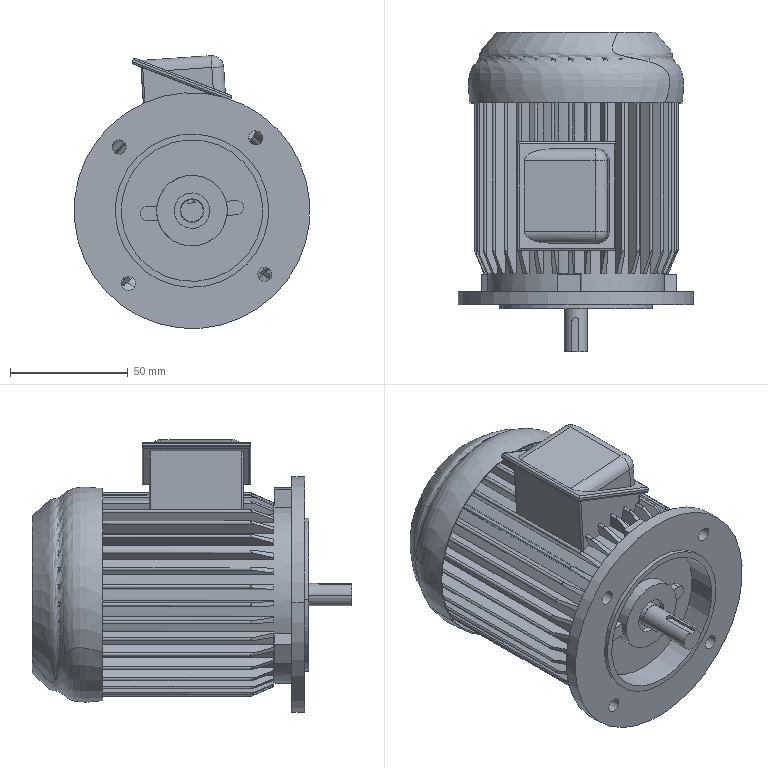Component | SolidWorks | Motor2-2 | 1 solid | 1244 faces | volume 547072 mm3 | plane 991 | cylinder 142 | cone 103 | spline 6 | sphere 2 | commonest cylinder face diameters 1.5 x72 6 x11 75 x11 10 x7 3.607 x4 2.865 x4 2.811 x4 4 x4